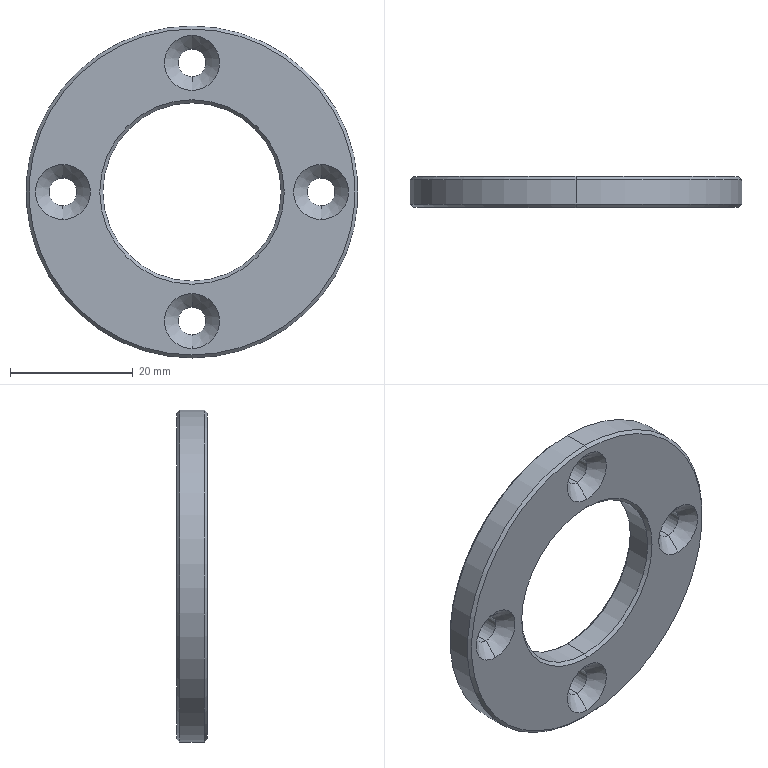Component | SolidWorks | ScrewRodBearingEndCap-1 | 1 solid | 30 faces | box 54 x 5 x 54 mm | volume 7578 mm3 | cone 16 | cylinder 12 | plane 2 | commonest cylinder face diameters 4.5 x8 29 x2 54 x2
build123d program:
from build123d import *

# Parameters (mm, degrees)
SKETCH1_R           = 27
SKETCH1_R_2         = 14.5
BOSS_EXTRUDE1_DEPTH = 5
CHAMFER1_SIZE       = 0.5
CIRPATTERN1_COUNT   = 4


with BuildPart() as part:
    # Sketch1 → Boss-Extrude1 (new body)
    with BuildSketch(Plane(origin=(0, 0, 0), x_dir=(1, 0, 0), z_dir=(0, 1, 0))):
        with Locations(Location((0, 0, 0), (0, 0, 270))):
            Circle(SKETCH1_R)
        with Locations(Location((0, 0, 0), (0, 0, 270))):
            Circle(SKETCH1_R_2, mode=Mode.SUBTRACT)
    extrude(amount=BOSS_EXTRUDE1_DEPTH)

    # Chamfer1
    chamfer1_edges = [part.edges().sort_by_distance(p)[0] for p in [
        (0, 0, -27),
        (0, 5, -27),
        (0, 0, -14.5),
        (0, 5, -14.5),
    ]]
    chamfer(chamfer1_edges, length=CHAMFER1_SIZE)

    # Sketch4 → M4 Hexagon Socket Countersunk Head Screw (revolve, cut)
    with BuildSketch(Plane(origin=(0, 0, 21), x_dir=(0, 0, -1), z_dir=(1, 0, 0))):
        Polygon((0, 0), (0, 16.352), (2.25, 15), (2.25, 2.23), (4.48, 0), align=None)
    m4_hexagon_socket_countersunk_head_screw = revolve(axis=Axis((0, -6.35, 21), (0, 1, 0)), mode=Mode.SUBTRACT)

    # CirPattern1: M4 Hexagon Socket Countersunk Head Screw ×4 about axis
    cirpattern1_axis = Axis((0, 0, 0), (0, 1, 0))
    for i in range(1, CIRPATTERN1_COUNT):
        add(m4_hexagon_socket_countersunk_head_screw.rotate(cirpattern1_axis, i * 360 / CIRPATTERN1_COUNT), mode=Mode.SUBTRACT)


solid = part.part

# Placed as in the assembly
solid = solid.moved(Location((-29.507, 212.589, 458), (0, 0, 0)))
STEP:
#1=COLOUR_RGB('',0.7922,0.8196,0.9333);
#2=FILL_AREA_STYLE_COLOUR('',#1);
#3=FILL_AREA_STYLE('',(#2));
#4=SURFACE_STYLE_FILL_AREA(#3);
#5=SURFACE_SIDE_STYLE('',(#4));
#6=SURFACE_STYLE_USAGE(.BOTH.,#5);
#7=PRESENTATION_STYLE_ASSIGNMENT((#6));
#8=CARTESIAN_POINT('',(-0.3349,8.457,18.12));
#9=VERTEX_POINT('',#8);
#10=CARTESIAN_POINT('',(-0.3349,8.457,17.943));
#11=VERTEX_POINT('',#10);
#12=CARTESIAN_POINT('',(-0.3349,8.457,18.031));
#13=DIRECTION('',(0.,-1.,0.));
#14=DIRECTION('',(0.,0.,-1.));
#15=AXIS2_PLACEMENT_3D('',#12,#13,#14);
#16=CIRCLE('',#15,0.08858);
#17=EDGE_CURVE('',#9,#11,#16,.T.);
#18=ORIENTED_EDGE('',*,*,#17,.F.);
#19=CARTESIAN_POINT('',(-0.3349,8.37,18.208));
#20=VERTEX_POINT('',#19);
#21=CARTESIAN_POINT('',(-0.3349,8.37,18.208));
#22=DIRECTION('',(0.,-0.7071,0.7071));
#23=VECTOR('',#22,39.37);
#24=LINE('',#21,#23);
#25=EDGE_CURVE('',#9,#20,#24,.T.);
#26=ORIENTED_EDGE('',*,*,#25,.T.);
#27=CARTESIAN_POINT('',(-0.3349,8.37,17.855));
#28=VERTEX_POINT('',#27);
#29=CARTESIAN_POINT('',(-0.3349,8.37,18.031));
#30=DIRECTION('',(0.,-1.,0.));
#31=DIRECTION('',(0.,0.,-1.));
#32=AXIS2_PLACEMENT_3D('',#29,#30,#31);
#33=CIRCLE('',#32,0.1764);
#34=EDGE_CURVE('',#20,#28,#33,.T.);
#35=ORIENTED_EDGE('',*,*,#34,.T.);
#36=CARTESIAN_POINT('',(-0.3349,8.37,17.855));
#37=DIRECTION('',(0.,-0.7071,-0.7071));
#38=VECTOR('',#37,39.37);
#39=LINE('',#36,#38);
#40=EDGE_CURVE('',#11,#28,#39,.T.);
#41=ORIENTED_EDGE('',*,*,#40,.F.);
#42=EDGE_LOOP('',(#18,#26,#35,#41));
#43=FACE_OUTER_BOUND('',#42,.T.);
#44=CARTESIAN_POINT('',(-0.3349,8.37,18.031));
#45=DIRECTION('',(0.,-1.,0.));
#46=DIRECTION('',(0.,0.,-1.));
#47=AXIS2_PLACEMENT_3D('',#44,#45,#46);
#48=CONICAL_SURFACE('',#47,0.1764,0.7854);
#49=ADVANCED_FACE('',(#43),#48,.F.);
#50=CARTESIAN_POINT('',(-0.3349,8.566,17.943));
#51=VERTEX_POINT('',#50);
#52=CARTESIAN_POINT('',(-0.3349,8.566,18.12));
#53=VERTEX_POINT('',#52);
#54=CARTESIAN_POINT('',(-0.3349,8.566,18.031));
#55=DIRECTION('',(0.,1.,0.));
#56=DIRECTION('',(0.,0.,1.));
#57=AXIS2_PLACEMENT_3D('',#54,#55,#56);
#58=CIRCLE('',#57,0.08858);
#59=EDGE_CURVE('',#51,#53,#58,.T.);
#60=ORIENTED_EDGE('',*,*,#59,.T.);
#61=CARTESIAN_POINT('',(-0.3349,8.37,18.12));
#62=DIRECTION('',(0.,-1.,0.));
#63=VECTOR('',#62,39.37);
#64=LINE('',#61,#63);
#65=EDGE_CURVE('',#53,#9,#64,.T.);
#66=ORIENTED_EDGE('',*,*,#65,.T.);
#67=ORIENTED_EDGE('',*,*,#17,.T.);
#68=CARTESIAN_POINT('',(-0.3349,8.37,17.943));
#69=DIRECTION('',(0.,-1.,0.));
#70=VECTOR('',#69,39.37);
#71=LINE('',#68,#70);
#72=EDGE_CURVE('',#51,#11,#71,.T.);
#73=ORIENTED_EDGE('',*,*,#72,.F.);
#74=EDGE_LOOP('',(#60,#66,#67,#73));
#75=FACE_OUTER_BOUND('',#74,.T.);
#76=CARTESIAN_POINT('',(-0.3349,8.37,18.031));
#77=DIRECTION('',(0.,-1.,0.));
#78=DIRECTION('',(0.,0.,-1.));
#79=AXIS2_PLACEMENT_3D('',#76,#77,#78);
#80=CYLINDRICAL_SURFACE('',#79,0.08858);
#81=ADVANCED_FACE('',(#75),#80,.F.);
#82=CARTESIAN_POINT('',(-1.162,8.457,17.293));
#83=VERTEX_POINT('',#82);
#84=CARTESIAN_POINT('',(-1.162,8.457,17.116));
#85=VERTEX_POINT('',#84);
#86=CARTESIAN_POINT('',(-1.162,8.457,17.205));
#87=DIRECTION('',(0.,-1.,0.));
#88=DIRECTION('',(0.,0.,-1.));
#89=AXIS2_PLACEMENT_3D('',#86,#87,#88);
#90=CIRCLE('',#89,0.08858);
#91=EDGE_CURVE('',#83,#85,#90,.T.);
#92=ORIENTED_EDGE('',*,*,#91,.F.);
#93=CARTESIAN_POINT('',(-1.162,8.37,17.381));
#94=VERTEX_POINT('',#93);
#95=CARTESIAN_POINT('',(-1.162,8.37,17.381));
#96=DIRECTION('',(0.,-0.7071,0.7071));
#97=VECTOR('',#96,39.37);
#98=LINE('',#95,#97);
#99=EDGE_CURVE('',#83,#94,#98,.T.);
#100=ORIENTED_EDGE('',*,*,#99,.T.);
#101=CARTESIAN_POINT('',(-1.162,8.37,17.028));
#102=VERTEX_POINT('',#101);
#103=CARTESIAN_POINT('',(-1.162,8.37,17.205));
#104=DIRECTION('',(0.,-1.,0.));
#105=DIRECTION('',(0.,0.,-1.));
#106=AXIS2_PLACEMENT_3D('',#103,#104,#105);
#107=CIRCLE('',#106,0.1764);
#108=EDGE_CURVE('',#94,#102,#107,.T.);
#109=ORIENTED_EDGE('',*,*,#108,.T.);
#110=CARTESIAN_POINT('',(-1.162,8.37,17.028));
#111=DIRECTION('',(0.,-0.7071,-0.7071));
#112=VECTOR('',#111,39.37);
#113=LINE('',#110,#112);
#114=EDGE_CURVE('',#85,#102,#113,.T.);
#115=ORIENTED_EDGE('',*,*,#114,.F.);
#116=EDGE_LOOP('',(#92,#100,#109,#115));
#117=FACE_OUTER_BOUND('',#116,.T.);
#118=CARTESIAN_POINT('',(-1.162,8.37,17.205));
#119=DIRECTION('',(0.,-1.,0.));
#120=DIRECTION('',(0.,0.,-1.));
#121=AXIS2_PLACEMENT_3D('',#118,#119,#120);
#122=CONICAL_SURFACE('',#121,0.1764,0.7854);
#123=ADVANCED_FACE('',(#117),#122,.F.);
#124=CARTESIAN_POINT('',(-1.162,8.566,17.116));
#125=VERTEX_POINT('',#124);
#126=CARTESIAN_POINT('',(-1.162,8.566,17.293));
#127=VERTEX_POINT('',#126);
#128=CARTESIAN_POINT('',(-1.162,8.566,17.205));
#129=DIRECTION('',(0.,1.,0.));
#130=DIRECTION('',(0.,0.,1.));
#131=AXIS2_PLACEMENT_3D('',#128,#129,#130);
#132=CIRCLE('',#131,0.08858);
#133=EDGE_CURVE('',#125,#127,#132,.T.);
#134=ORIENTED_EDGE('',*,*,#133,.T.);
#135=CARTESIAN_POINT('',(-1.162,8.37,17.293));
#136=DIRECTION('',(0.,-1.,0.));
#137=VECTOR('',#136,39.37);
#138=LINE('',#135,#137);
#139=EDGE_CURVE('',#127,#83,#138,.T.);
#140=ORIENTED_EDGE('',*,*,#139,.T.);
#141=ORIENTED_EDGE('',*,*,#91,.T.);
#142=CARTESIAN_POINT('',(-1.162,8.37,17.116));
#143=DIRECTION('',(0.,-1.,0.));
#144=VECTOR('',#143,39.37);
#145=LINE('',#142,#144);
#146=EDGE_CURVE('',#125,#85,#145,.T.);
#147=ORIENTED_EDGE('',*,*,#146,.F.);
#148=EDGE_LOOP('',(#134,#140,#141,#147));
#149=FACE_OUTER_BOUND('',#148,.T.);
#150=CARTESIAN_POINT('',(-1.162,8.37,17.205));
#151=DIRECTION('',(0.,-1.,0.));
#152=DIRECTION('',(0.,0.,-1.));
#153=AXIS2_PLACEMENT_3D('',#150,#151,#152);
#154=CYLINDRICAL_SURFACE('',#153,0.08858);
#155=ADVANCED_FACE('',(#149),#154,.F.);
#156=CARTESIAN_POINT('',(-1.988,8.457,18.12));
#157=VERTEX_POINT('',#156);
#158=CARTESIAN_POINT('',(-1.988,8.457,17.943));
#159=VERTEX_POINT('',#158);
#160=CARTESIAN_POINT('',(-1.988,8.457,18.031));
#161=DIRECTION('',(0.,-1.,0.));
#162=DIRECTION('',(0.,0.,-1.));
#163=AXIS2_PLACEMENT_3D('',#160,#161,#162);
#164=CIRCLE('',#163,0.08858);
#165=EDGE_CURVE('',#157,#159,#164,.T.);
#166=ORIENTED_EDGE('',*,*,#165,.F.);
#167=CARTESIAN_POINT('',(-1.988,8.37,18.208));
#168=VERTEX_POINT('',#167);
#169=CARTESIAN_POINT('',(-1.988,8.37,18.208));
#170=DIRECTION('',(0.,-0.7071,0.7071));
#171=VECTOR('',#170,39.37);
#172=LINE('',#169,#171);
#173=EDGE_CURVE('',#157,#168,#172,.T.);
#174=ORIENTED_EDGE('',*,*,#173,.T.);
#175=CARTESIAN_POINT('',(-1.988,8.37,17.855));
#176=VERTEX_POINT('',#175);
#177=CARTESIAN_POINT('',(-1.988,8.37,18.031));
#178=DIRECTION('',(0.,-1.,0.));
#179=DIRECTION('',(0.,0.,-1.));
#180=AXIS2_PLACEMENT_3D('',#177,#178,#179);
#181=CIRCLE('',#180,0.1764);
#182=EDGE_CURVE('',#168,#176,#181,.T.);
#183=ORIENTED_EDGE('',*,*,#182,.T.);
#184=CARTESIAN_POINT('',(-1.988,8.37,17.855));
#185=DIRECTION('',(0.,-0.7071,-0.7071));
#186=VECTOR('',#185,39.37);
#187=LINE('',#184,#186);
#188=EDGE_CURVE('',#159,#176,#187,.T.);
#189=ORIENTED_EDGE('',*,*,#188,.F.);
#190=EDGE_LOOP('',(#166,#174,#183,#189));
#191=FACE_OUTER_BOUND('',#190,.T.);
#192=CARTESIAN_POINT('',(-1.988,8.37,18.031));
#193=DIRECTION('',(0.,-1.,0.));
#194=DIRECTION('',(0.,0.,-1.));
#195=AXIS2_PLACEMENT_3D('',#192,#193,#194);
#196=CONICAL_SURFACE('',#195,0.1764,0.7854);
#197=ADVANCED_FACE('',(#191),#196,.F.);
#198=CARTESIAN_POINT('',(-1.988,8.566,17.943));
#199=VERTEX_POINT('',#198);
#200=CARTESIAN_POINT('',(-1.988,8.566,18.12));
#201=VERTEX_POINT('',#200);
#202=CARTESIAN_POINT('',(-1.988,8.566,18.031));
#203=DIRECTION('',(0.,1.,0.));
#204=DIRECTION('',(0.,0.,1.));
#205=AXIS2_PLACEMENT_3D('',#202,#203,#204);
#206=CIRCLE('',#205,0.08858);
#207=EDGE_CURVE('',#199,#201,#206,.T.);
#208=ORIENTED_EDGE('',*,*,#207,.T.);
#209=CARTESIAN_POINT('',(-1.988,8.37,18.12));
#210=DIRECTION('',(0.,-1.,0.));
#211=VECTOR('',#210,39.37);
#212=LINE('',#209,#211);
#213=EDGE_CURVE('',#201,#157,#212,.T.);
#214=ORIENTED_EDGE('',*,*,#213,.T.);
#215=ORIENTED_EDGE('',*,*,#165,.T.);
#216=CARTESIAN_POINT('',(-1.988,8.37,17.943));
#217=DIRECTION('',(0.,-1.,0.));
#218=VECTOR('',#217,39.37);
#219=LINE('',#216,#218);
#220=EDGE_CURVE('',#199,#159,#219,.T.);
#221=ORIENTED_EDGE('',*,*,#220,.F.);
#222=EDGE_LOOP('',(#208,#214,#215,#221));
#223=FACE_OUTER_BOUND('',#222,.T.);
#224=CARTESIAN_POINT('',(-1.988,8.37,18.031));
#225=DIRECTION('',(0.,-1.,0.));
#226=DIRECTION('',(0.,0.,-1.));
#227=AXIS2_PLACEMENT_3D('',#224,#225,#226);
#228=CYLINDRICAL_SURFACE('',#227,0.08858);
#229=ADVANCED_FACE('',(#223),#228,.F.);
#230=CARTESIAN_POINT('',(-1.162,8.457,18.947));
#231=VERTEX_POINT('',#230);
#232=CARTESIAN_POINT('',(-1.162,8.457,18.77));
#233=VERTEX_POINT('',#232);
#234=CARTESIAN_POINT('',(-1.162,8.457,18.858));
#235=DIRECTION('',(0.,-1.,0.));
#236=DIRECTION('',(0.,0.,-1.));
#237=AXIS2_PLACEMENT_3D('',#234,#235,#236);
#238=CIRCLE('',#237,0.08858);
#239=EDGE_CURVE('',#231,#233,#238,.T.);
#240=ORIENTED_EDGE('',*,*,#239,.F.);
#241=CARTESIAN_POINT('',(-1.162,8.37,19.035));
#242=VERTEX_POINT('',#241);
#243=CARTESIAN_POINT('',(-1.162,8.37,19.035));
#244=DIRECTION('',(0.,-0.7071,0.7071));
#245=VECTOR('',#244,39.37);
#246=LINE('',#243,#245);
#247=EDGE_CURVE('',#231,#242,#246,.T.);
#248=ORIENTED_EDGE('',*,*,#247,.T.);
#249=CARTESIAN_POINT('',(-1.162,8.37,18.682));
#250=VERTEX_POINT('',#249);
#251=CARTESIAN_POINT('',(-1.162,8.37,18.858));
#252=DIRECTION('',(0.,-1.,0.));
#253=DIRECTION('',(0.,0.,-1.));
#254=AXIS2_PLACEMENT_3D('',#251,#252,#253);
#255=CIRCLE('',#254,0.1764);
#256=EDGE_CURVE('',#242,#250,#255,.T.);
#257=ORIENTED_EDGE('',*,*,#256,.T.);
#258=CARTESIAN_POINT('',(-1.162,8.37,18.682));
#259=DIRECTION('',(0.,-0.7071,-0.7071));
#260=VECTOR('',#259,39.37);
#261=LINE('',#258,#260);
#262=EDGE_CURVE('',#233,#250,#261,.T.);
#263=ORIENTED_EDGE('',*,*,#262,.F.);
#264=EDGE_LOOP('',(#240,#248,#257,#263));
#265=FACE_OUTER_BOUND('',#264,.T.);
#266=CARTESIAN_POINT('',(-1.162,8.37,18.858));
#267=DIRECTION('',(0.,-1.,0.));
#268=DIRECTION('',(0.,0.,-1.));
#269=AXIS2_PLACEMENT_3D('',#266,#267,#268);
#270=CONICAL_SURFACE('',#269,0.1764,0.7854);
#271=ADVANCED_FACE('',(#265),#270,.F.);
#272=CARTESIAN_POINT('',(-1.162,8.566,18.77));
#273=VERTEX_POINT('',#272);
#274=CARTESIAN_POINT('',(-1.162,8.566,18.947));
#275=VERTEX_POINT('',#274);
#276=CARTESIAN_POINT('',(-1.162,8.566,18.858));
#277=DIRECTION('',(0.,1.,0.));
#278=DIRECTION('',(0.,0.,1.));
#279=AXIS2_PLACEMENT_3D('',#276,#277,#278);
#280=CIRCLE('',#279,0.08858);
#281=EDGE_CURVE('',#273,#275,#280,.T.);
#282=ORIENTED_EDGE('',*,*,#281,.T.);
#283=CARTESIAN_POINT('',(-1.162,8.37,18.947));
#284=DIRECTION('',(0.,-1.,0.));
#285=VECTOR('',#284,39.37);
#286=LINE('',#283,#285);
#287=EDGE_CURVE('',#275,#231,#286,.T.);
#288=ORIENTED_EDGE('',*,*,#287,.T.);
#289=ORIENTED_EDGE('',*,*,#239,.T.);
#290=CARTESIAN_POINT('',(-1.162,8.37,18.77));
#291=DIRECTION('',(0.,-1.,0.));
#292=VECTOR('',#291,39.37);
#293=LINE('',#290,#292);
#294=EDGE_CURVE('',#273,#233,#293,.T.);
#295=ORIENTED_EDGE('',*,*,#294,.F.);
#296=EDGE_LOOP('',(#282,#288,#289,#295));
#297=FACE_OUTER_BOUND('',#296,.T.);
#298=CARTESIAN_POINT('',(-1.162,8.37,18.858));
#299=DIRECTION('',(0.,-1.,0.));
#300=DIRECTION('',(0.,0.,-1.));
#301=AXIS2_PLACEMENT_3D('',#298,#299,#300);
#302=CYLINDRICAL_SURFACE('',#301,0.08858);
#303=ADVANCED_FACE('',(#297),#302,.F.);
#304=CARTESIAN_POINT('',(-1.162,8.547,17.461));
#305=VERTEX_POINT('',#304);
#306=CARTESIAN_POINT('',(-1.162,8.547,18.602));
#307=VERTEX_POINT('',#306);
#308=CARTESIAN_POINT('',(-1.162,8.547,18.031));
#309=DIRECTION('',(0.,1.,0.));
#310=DIRECTION('',(0.,0.,1.));
#311=AXIS2_PLACEMENT_3D('',#308,#309,#310);
#312=CIRCLE('',#311,0.5709);
#313=EDGE_CURVE('',#305,#307,#312,.T.);
#314=ORIENTED_EDGE('',*,*,#313,.F.);
#315=CARTESIAN_POINT('',(-1.162,8.566,17.441));
#316=VERTEX_POINT('',#315);
#317=CARTESIAN_POINT('',(-1.162,8.547,17.461));
#318=DIRECTION('',(0.,0.7071,-0.7071));
#319=VECTOR('',#318,39.37);
#320=LINE('',#317,#319);
#321=EDGE_CURVE('',#305,#316,#320,.T.);
#322=ORIENTED_EDGE('',*,*,#321,.T.);
#323=CARTESIAN_POINT('',(-1.162,8.566,18.622));
#324=VERTEX_POINT('',#323);
#325=CARTESIAN_POINT('',(-1.162,8.566,18.031));
#326=DIRECTION('',(0.,-1.,0.));
#327=DIRECTION('',(0.,0.,1.));
#328=AXIS2_PLACEMENT_3D('',#325,#326,#327);
#329=CIRCLE('',#328,0.5906);
#330=EDGE_CURVE('',#324,#316,#329,.T.);
#331=ORIENTED_EDGE('',*,*,#330,.F.);
#332=CARTESIAN_POINT('',(-1.162,8.547,18.602));
#333=DIRECTION('',(0.,0.7071,0.7071));
#334=VECTOR('',#333,39.37);
#335=LINE('',#332,#334);
#336=EDGE_CURVE('',#307,#324,#335,.T.);
#337=ORIENTED_EDGE('',*,*,#336,.F.);
#338=EDGE_LOOP('',(#314,#322,#331,#337));
#339=FACE_OUTER_BOUND('',#338,.T.);
#340=CARTESIAN_POINT('',(-1.162,8.547,18.031));
#341=DIRECTION('',(0.,1.,0.));
#342=DIRECTION('',(0.,0.,1.));
#343=AXIS2_PLACEMENT_3D('',#340,#341,#342);
#344=CONICAL_SURFACE('',#343,0.5709,0.7854);
#345=ADVANCED_FACE('',(#339),#344,.F.);
#346=CARTESIAN_POINT('',(-1.162,8.566,19.075));
#347=VERTEX_POINT('',#346);
#348=CARTESIAN_POINT('',(-1.162,8.566,16.988));
#349=VERTEX_POINT('',#348);
#350=CARTESIAN_POINT('',(-1.162,8.566,18.031));
#351=DIRECTION('',(0.,1.,0.));
#352=DIRECTION('',(0.,0.,1.));
#353=AXIS2_PLACEMENT_3D('',#350,#351,#352);
#354=CIRCLE('',#353,1.043);
#355=EDGE_CURVE('',#347,#349,#354,.T.);
#356=ORIENTED_EDGE('',*,*,#355,.F.);
#357=CARTESIAN_POINT('',(-1.162,8.547,19.094));
#358=VERTEX_POINT('',#357);
#359=CARTESIAN_POINT('',(-1.162,8.566,19.075));
#360=DIRECTION('',(0.,-0.7071,0.7071));
#361=VECTOR('',#360,39.37);
#362=LINE('',#359,#361);
#363=EDGE_CURVE('',#347,#358,#362,.T.);
#364=ORIENTED_EDGE('',*,*,#363,.T.);
#365=CARTESIAN_POINT('',(-1.162,8.547,16.969));
#366=VERTEX_POINT('',#365);
#367=CARTESIAN_POINT('',(-1.162,8.547,18.031));
#368=DIRECTION('',(0.,-1.,0.));
#369=DIRECTION('',(0.,0.,1.));
#370=AXIS2_PLACEMENT_3D('',#367,#368,#369);
#371=CIRCLE('',#370,1.063);
#372=EDGE_CURVE('',#366,#358,#371,.T.);
#373=ORIENTED_EDGE('',*,*,#372,.F.);
#374=CARTESIAN_POINT('',(-1.162,8.566,16.988));
#375=DIRECTION('',(0.,-0.7071,-0.7071));
#376=VECTOR('',#375,39.37);
#377=LINE('',#374,#376);
#378=EDGE_CURVE('',#349,#366,#377,.T.);
#379=ORIENTED_EDGE('',*,*,#378,.F.);
#380=EDGE_LOOP('',(#356,#364,#373,#379));
#381=FACE_OUTER_BOUND('',#380,.T.);
#382=CARTESIAN_POINT('',(-1.162,8.566,18.031));
#383=DIRECTION('',(0.,-1.,0.));
#384=DIRECTION('',(0.,0.,-1.));
#385=AXIS2_PLACEMENT_3D('',#382,#383,#384);
#386=CONICAL_SURFACE('',#385,1.043,0.7854);
#387=ADVANCED_FACE('',(#381),#386,.T.);
#388=CARTESIAN_POINT('',(-1.162,8.37,16.988));
#389=VERTEX_POINT('',#388);
#390=CARTESIAN_POINT('',(-1.162,8.37,19.075));
#391=VERTEX_POINT('',#390);
#392=CARTESIAN_POINT('',(-1.162,8.37,18.031));
#393=DIRECTION('',(0.,-1.,0.));
#394=DIRECTION('',(0.,0.,1.));
#395=AXIS2_PLACEMENT_3D('',#392,#393,#394);
#396=CIRCLE('',#395,1.043);
#397=EDGE_CURVE('',#389,#391,#396,.T.);
#398=ORIENTED_EDGE('',*,*,#397,.F.);
#399=CARTESIAN_POINT('',(-1.162,8.389,16.969));
#400=VERTEX_POINT('',#399);
#401=CARTESIAN_POINT('',(-1.162,8.389,16.969));
#402=DIRECTION('',(0.,0.7071,-0.7071));
#403=VECTOR('',#402,39.37);
#404=LINE('',#401,#403);
#405=EDGE_CURVE('',#389,#400,#404,.T.);
#406=ORIENTED_EDGE('',*,*,#405,.T.);
#407=CARTESIAN_POINT('',(-1.162,8.389,19.094));
#408=VERTEX_POINT('',#407);
#409=CARTESIAN_POINT('',(-1.162,8.389,18.031));
#410=DIRECTION('',(0.,1.,0.));
#411=DIRECTION('',(0.,0.,1.));
#412=AXIS2_PLACEMENT_3D('',#409,#410,#411);
#413=CIRCLE('',#412,1.063);
#414=EDGE_CURVE('',#408,#400,#413,.T.);
#415=ORIENTED_EDGE('',*,*,#414,.F.);
#416=CARTESIAN_POINT('',(-1.162,8.389,19.094));
#417=DIRECTION('',(0.,0.7071,0.7071));
#418=VECTOR('',#417,39.37);
#419=LINE('',#416,#418);
#420=EDGE_CURVE('',#391,#408,#419,.T.);
#421=ORIENTED_EDGE('',*,*,#420,.F.);
#422=EDGE_LOOP('',(#398,#406,#415,#421));
#423=FACE_OUTER_BOUND('',#422,.T.);
#424=CARTESIAN_POINT('',(-1.162,8.389,18.031));
#425=DIRECTION('',(0.,1.,0.));
#426=DIRECTION('',(0.,0.,1.));
#427=AXIS2_PLACEMENT_3D('',#424,#425,#426);
#428=CONICAL_SURFACE('',#427,1.063,0.7854);
#429=ADVANCED_FACE('',(#423),#428,.T.);
#430=CARTESIAN_POINT('',(-1.162,8.389,18.602));
#431=VERTEX_POINT('',#430);
#432=CARTESIAN_POINT('',(-1.162,8.389,17.461));
#433=VERTEX_POINT('',#432);
#434=CARTESIAN_POINT('',(-1.162,8.389,18.031));
#435=DIRECTION('',(0.,-1.,0.));
#436=DIRECTION('',(0.,0.,1.));
#437=AXIS2_PLACEMENT_3D('',#434,#435,#436);
#438=CIRCLE('',#437,0.5709);
#439=EDGE_CURVE('',#431,#433,#438,.T.);
#440=ORIENTED_EDGE('',*,*,#439,.F.);
#441=CARTESIAN_POINT('',(-1.162,8.37,18.622));
#442=VERTEX_POINT('',#441);
#443=CARTESIAN_POINT('',(-1.162,8.37,18.622));
#444=DIRECTION('',(0.,-0.7071,0.7071));
#445=VECTOR('',#444,39.37);
#446=LINE('',#443,#445);
#447=EDGE_CURVE('',#431,#442,#446,.T.);
#448=ORIENTED_EDGE('',*,*,#447,.T.);
#449=CARTESIAN_POINT('',(-1.162,8.37,17.441));
#450=VERTEX_POINT('',#449);
#451=CARTESIAN_POINT('',(-1.162,8.37,18.031));
#452=DIRECTION('',(0.,1.,0.));
#453=DIRECTION('',(0.,0.,1.));
#454=AXIS2_PLACEMENT_3D('',#451,#452,#453);
#455=CIRCLE('',#454,0.5906);
#456=EDGE_CURVE('',#450,#442,#455,.T.);
#457=ORIENTED_EDGE('',*,*,#456,.F.);
#458=CARTESIAN_POINT('',(-1.162,8.37,17.441));
#459=DIRECTION('',(0.,-0.7071,-0.7071));
#460=VECTOR('',#459,39.37);
#461=LINE('',#458,#460);
#462=EDGE_CURVE('',#433,#450,#461,.T.);
#463=ORIENTED_EDGE('',*,*,#462,.F.);
#464=EDGE_LOOP('',(#440,#448,#457,#463));
#465=FACE_OUTER_BOUND('',#464,.T.);
#466=CARTESIAN_POINT('',(-1.162,8.37,18.031));
#467=DIRECTION('',(0.,-1.,0.));
#468=DIRECTION('',(0.,0.,-1.));
#469=AXIS2_PLACEMENT_3D('',#466,#467,#468);
#470=CONICAL_SURFACE('',#469,0.5906,0.7854);
#471=ADVANCED_FACE('',(#465),#470,.F.);
#472=ORIENTED_EDGE('',*,*,#313,.T.);
#473=CARTESIAN_POINT('',(-1.162,8.566,18.602));
#474=DIRECTION('',(0.,-1.,0.));
#475=VECTOR('',#474,39.37);
#476=LINE('',#473,#475);
#477=EDGE_CURVE('',#307,#431,#476,.T.);
#478=ORIENTED_EDGE('',*,*,#477,.T.);
#479=ORIENTED_EDGE('',*,*,#439,.T.);
#480=CARTESIAN_POINT('',(-1.162,8.566,17.461));
#481=DIRECTION('',(0.,-1.,0.));
#482=VECTOR('',#481,39.37);
#483=LINE('',#480,#482);
#484=EDGE_CURVE('',#305,#433,#483,.T.);
#485=ORIENTED_EDGE('',*,*,#484,.F.);
#486=EDGE_LOOP('',(#472,#478,#479,#485));
#487=FACE_OUTER_BOUND('',#486,.T.);
#488=CARTESIAN_POINT('',(-1.162,8.566,18.031));
#489=DIRECTION('',(0.,-1.,0.));
#490=DIRECTION('',(0.,0.,-1.));
#491=AXIS2_PLACEMENT_3D('',#488,#489,#490);
#492=CYLINDRICAL_SURFACE('',#491,0.5709);
#493=ADVANCED_FACE('',(#487),#492,.F.);
#494=ORIENTED_EDGE('',*,*,#372,.T.);
#495=CARTESIAN_POINT('',(-1.162,8.566,19.094));
#496=DIRECTION('',(0.,-1.,0.));
#497=VECTOR('',#496,39.37);
#498=LINE('',#495,#497);
#499=EDGE_CURVE('',#358,#408,#498,.T.);
#500=ORIENTED_EDGE('',*,*,#499,.T.);
#501=ORIENTED_EDGE('',*,*,#414,.T.);
#502=CARTESIAN_POINT('',(-1.162,8.566,16.969));
#503=DIRECTION('',(0.,-1.,0.));
#504=VECTOR('',#503,39.37);
#505=LINE('',#502,#504);
#506=EDGE_CURVE('',#366,#400,#505,.T.);
#507=ORIENTED_EDGE('',*,*,#506,.F.);
#508=EDGE_LOOP('',(#494,#500,#501,#507));
#509=FACE_OUTER_BOUND('',#508,.T.);
#510=CARTESIAN_POINT('',(-1.162,8.566,18.031));
#511=DIRECTION('',(0.,-1.,0.));
#512=DIRECTION('',(0.,0.,-1.));
#513=AXIS2_PLACEMENT_3D('',#510,#511,#512);
#514=CYLINDRICAL_SURFACE('',#513,1.063);
#515=ADVANCED_FACE('',(#509),#514,.T.);
#516=ORIENTED_EDGE('',*,*,#59,.F.);
#517=CARTESIAN_POINT('',(-0.3349,8.566,18.031));
#518=DIRECTION('',(0.,1.,0.));
#519=DIRECTION('',(0.,0.,1.));
#520=AXIS2_PLACEMENT_3D('',#517,#518,#519);
#521=CIRCLE('',#520,0.08858);
#522=EDGE_CURVE('',#53,#51,#521,.T.);
#523=ORIENTED_EDGE('',*,*,#522,.F.);
#524=EDGE_LOOP('',(#516,#523));
#525=FACE_BOUND('',#524,.T.);
#526=ORIENTED_EDGE('',*,*,#133,.F.);
#527=CARTESIAN_POINT('',(-1.162,8.566,17.205));
#528=DIRECTION('',(0.,1.,0.));
#529=DIRECTION('',(0.,0.,1.));
#530=AXIS2_PLACEMENT_3D('',#527,#528,#529);
#531=CIRCLE('',#530,0.08858);
#532=EDGE_CURVE('',#127,#125,#531,.T.);
#533=ORIENTED_EDGE('',*,*,#532,.F.);
#534=EDGE_LOOP('',(#526,#533));
#535=FACE_BOUND('',#534,.T.);
#536=ORIENTED_EDGE('',*,*,#207,.F.);
#537=CARTESIAN_POINT('',(-1.988,8.566,18.031));
#538=DIRECTION('',(0.,1.,0.));
#539=DIRECTION('',(0.,0.,1.));
#540=AXIS2_PLACEMENT_3D('',#537,#538,#539);
#541=CIRCLE('',#540,0.08858);
#542=EDGE_CURVE('',#201,#199,#541,.T.);
#543=ORIENTED_EDGE('',*,*,#542,.F.);
#544=EDGE_LOOP('',(#536,#543));
#545=FACE_BOUND('',#544,.T.);
#546=ORIENTED_EDGE('',*,*,#281,.F.);
#547=CARTESIAN_POINT('',(-1.162,8.566,18.858));
#548=DIRECTION('',(0.,1.,0.));
#549=DIRECTION('',(0.,0.,1.));
#550=AXIS2_PLACEMENT_3D('',#547,#548,#549);
#551=CIRCLE('',#550,0.08858);
#552=EDGE_CURVE('',#275,#273,#551,.T.);
#553=ORIENTED_EDGE('',*,*,#552,.F.);
#554=EDGE_LOOP('',(#546,#553));
#555=FACE_BOUND('',#554,.T.);
#556=CARTESIAN_POINT('',(-1.162,8.566,18.031));
#557=DIRECTION('',(0.,1.,0.));
#558=DIRECTION('',(0.,0.,1.));
#559=AXIS2_PLACEMENT_3D('',#556,#557,#558);
#560=CIRCLE('',#559,1.043);
#561=EDGE_CURVE('',#349,#347,#560,.T.);
#562=ORIENTED_EDGE('',*,*,#561,.T.);
#563=ORIENTED_EDGE('',*,*,#355,.T.);
#564=EDGE_LOOP('',(#562,#563));
#565=FACE_OUTER_BOUND('',#564,.T.);
#566=ORIENTED_EDGE('',*,*,#330,.T.);
#567=CARTESIAN_POINT('',(-1.162,8.566,18.031));
#568=DIRECTION('',(0.,-1.,0.));
#569=DIRECTION('',(0.,0.,1.));
#570=AXIS2_PLACEMENT_3D('',#567,#568,#569);
#571=CIRCLE('',#570,0.5906);
#572=EDGE_CURVE('',#316,#324,#571,.T.);
#573=ORIENTED_EDGE('',*,*,#572,.T.);
#574=EDGE_LOOP('',(#566,#573));
#575=FACE_BOUND('',#574,.T.);
#576=CARTESIAN_POINT('',(-1.162,8.566,18.031));
#577=DIRECTION('',(0.,1.,0.));
#578=DIRECTION('',(0.,0.,1.));
#579=AXIS2_PLACEMENT_3D('',#576,#577,#578);
#580=PLANE('',#579);
#581=ADVANCED_FACE('',(#525,#535,#545,#555,#565,#575),#580,.T.);
#582=CARTESIAN_POINT('',(-0.3349,8.37,18.031));
#583=DIRECTION('',(0.,-1.,0.));
#584=DIRECTION('',(0.,0.,-1.));
#585=AXIS2_PLACEMENT_3D('',#582,#583,#584);
#586=CIRCLE('',#585,0.1764);
#587=EDGE_CURVE('',#28,#20,#586,.T.);
#588=ORIENTED_EDGE('',*,*,#587,.F.);
#589=ORIENTED_EDGE('',*,*,#34,.F.);
#590=EDGE_LOOP('',(#588,#589));
#591=FACE_BOUND('',#590,.T.);
#592=CARTESIAN_POINT('',(-1.162,8.37,17.205));
#593=DIRECTION('',(0.,-1.,0.));
#594=DIRECTION('',(0.,0.,-1.));
#595=AXIS2_PLACEMENT_3D('',#592,#593,#594);
#596=CIRCLE('',#595,0.1764);
#597=EDGE_CURVE('',#102,#94,#596,.T.);
#598=ORIENTED_EDGE('',*,*,#597,.F.);
#599=ORIENTED_EDGE('',*,*,#108,.F.);
#600=EDGE_LOOP('',(#598,#599));
#601=FACE_BOUND('',#600,.T.);
#602=CARTESIAN_POINT('',(-1.988,8.37,18.031));
#603=DIRECTION('',(0.,-1.,0.));
#604=DIRECTION('',(0.,0.,-1.));
#605=AXIS2_PLACEMENT_3D('',#602,#603,#604);
#606=CIRCLE('',#605,0.1764);
#607=EDGE_CURVE('',#176,#168,#606,.T.);
#608=ORIENTED_EDGE('',*,*,#607,.F.);
#609=ORIENTED_EDGE('',*,*,#182,.F.);
#610=EDGE_LOOP('',(#608,#609));
#611=FACE_BOUND('',#610,.T.);
#612=CARTESIAN_POINT('',(-1.162,8.37,18.858));
#613=DIRECTION('',(0.,-1.,0.));
#614=DIRECTION('',(0.,0.,-1.));
#615=AXIS2_PLACEMENT_3D('',#612,#613,#614);
#616=CIRCLE('',#615,0.1764);
#617=EDGE_CURVE('',#250,#242,#616,.T.);
#618=ORIENTED_EDGE('',*,*,#617,.F.);
#619=ORIENTED_EDGE('',*,*,#256,.F.);
#620=EDGE_LOOP('',(#618,#619));
#621=FACE_BOUND('',#620,.T.);
#622=ORIENTED_EDGE('',*,*,#456,.T.);
#623=CARTESIAN_POINT('',(-1.162,8.37,18.031));
#624=DIRECTION('',(0.,1.,0.));
#625=DIRECTION('',(0.,0.,1.));
#626=AXIS2_PLACEMENT_3D('',#623,#624,#625);
#627=CIRCLE('',#626,0.5906);
#628=EDGE_CURVE('',#442,#450,#627,.T.);
#629=ORIENTED_EDGE('',*,*,#628,.T.);
#630=EDGE_LOOP('',(#622,#629));
#631=FACE_BOUND('',#630,.T.);
#632=CARTESIAN_POINT('',(-1.162,8.37,18.031));
#633=DIRECTION('',(0.,-1.,0.));
#634=DIRECTION('',(0.,0.,1.));
#635=AXIS2_PLACEMENT_3D('',#632,#633,#634);
#636=CIRCLE('',#635,1.043);
#637=EDGE_CURVE('',#391,#389,#636,.T.);
#638=ORIENTED_EDGE('',*,*,#637,.T.);
#639=ORIENTED_EDGE('',*,*,#397,.T.);
#640=EDGE_LOOP('',(#638,#639));
#641=FACE_OUTER_BOUND('',#640,.T.);
#642=CARTESIAN_POINT('',(-1.162,8.37,18.031));
#643=DIRECTION('',(0.,1.,0.));
#644=DIRECTION('',(0.,0.,1.));
#645=AXIS2_PLACEMENT_3D('',#642,#643,#644);
#646=PLANE('',#645);
#647=ADVANCED_FACE('',(#591,#601,#611,#621,#631,#641),#646,.F.);
#648=ORIENTED_EDGE('',*,*,#499,.F.);
#649=CARTESIAN_POINT('',(-1.162,8.547,18.031));
#650=DIRECTION('',(0.,-1.,0.));
#651=DIRECTION('',(0.,0.,1.));
#652=AXIS2_PLACEMENT_3D('',#649,#650,#651);
#653=CIRCLE('',#652,1.063);
#654=EDGE_CURVE('',#358,#366,#653,.T.);
#655=ORIENTED_EDGE('',*,*,#654,.T.);
#656=ORIENTED_EDGE('',*,*,#506,.T.);
#657=CARTESIAN_POINT('',(-1.162,8.389,18.031));
#658=DIRECTION('',(0.,1.,0.));
#659=DIRECTION('',(0.,0.,1.));
#660=AXIS2_PLACEMENT_3D('',#657,#658,#659);
#661=CIRCLE('',#660,1.063);
#662=EDGE_CURVE('',#400,#408,#661,.T.);
#663=ORIENTED_EDGE('',*,*,#662,.T.);
#664=EDGE_LOOP('',(#648,#655,#656,#663));
#665=FACE_OUTER_BOUND('',#664,.T.);
#666=CARTESIAN_POINT('',(-1.162,8.566,18.031));
#667=DIRECTION('',(0.,-1.,0.));
#668=DIRECTION('',(0.,0.,-1.));
#669=AXIS2_PLACEMENT_3D('',#666,#667,#668);
#670=CYLINDRICAL_SURFACE('',#669,1.063);
#671=ADVANCED_FACE('',(#665),#670,.T.);
#672=ORIENTED_EDGE('',*,*,#477,.F.);
#673=CARTESIAN_POINT('',(-1.162,8.547,18.031));
#674=DIRECTION('',(0.,1.,0.));
#675=DIRECTION('',(0.,0.,1.));
#676=AXIS2_PLACEMENT_3D('',#673,#674,#675);
#677=CIRCLE('',#676,0.5709);
#678=EDGE_CURVE('',#307,#305,#677,.T.);
#679=ORIENTED_EDGE('',*,*,#678,.T.);
#680=ORIENTED_EDGE('',*,*,#484,.T.);
#681=CARTESIAN_POINT('',(-1.162,8.389,18.031));
#682=DIRECTION('',(0.,-1.,0.));
#683=DIRECTION('',(0.,0.,1.));
#684=AXIS2_PLACEMENT_3D('',#681,#682,#683);
#685=CIRCLE('',#684,0.5709);
#686=EDGE_CURVE('',#433,#431,#685,.T.);
#687=ORIENTED_EDGE('',*,*,#686,.T.);
#688=EDGE_LOOP('',(#672,#679,#680,#687));
#689=FACE_OUTER_BOUND('',#688,.T.);
#690=CARTESIAN_POINT('',(-1.162,8.566,18.031));
#691=DIRECTION('',(0.,-1.,0.));
#692=DIRECTION('',(0.,0.,-1.));
#693=AXIS2_PLACEMENT_3D('',#690,#691,#692);
#694=CYLINDRICAL_SURFACE('',#693,0.5709);
#695=ADVANCED_FACE('',(#689),#694,.F.);
#696=ORIENTED_EDGE('',*,*,#447,.F.);
#697=ORIENTED_EDGE('',*,*,#686,.F.);
#698=ORIENTED_EDGE('',*,*,#462,.T.);
#699=ORIENTED_EDGE('',*,*,#628,.F.);
#700=EDGE_LOOP('',(#696,#697,#698,#699));
#701=FACE_OUTER_BOUND('',#700,.T.);
#702=CARTESIAN_POINT('',(-1.162,8.37,18.031));
#703=DIRECTION('',(0.,-1.,0.));
#704=DIRECTION('',(0.,0.,-1.));
#705=AXIS2_PLACEMENT_3D('',#702,#703,#704);
#706=CONICAL_SURFACE('',#705,0.5906,0.7854);
#707=ADVANCED_FACE('',(#701),#706,.F.);
#708=ORIENTED_EDGE('',*,*,#405,.F.);
#709=ORIENTED_EDGE('',*,*,#637,.F.);
#710=ORIENTED_EDGE('',*,*,#420,.T.);
#711=ORIENTED_EDGE('',*,*,#662,.F.);
#712=EDGE_LOOP('',(#708,#709,#710,#711));
#713=FACE_OUTER_BOUND('',#712,.T.);
#714=CARTESIAN_POINT('',(-1.162,8.389,18.031));
#715=DIRECTION('',(0.,1.,0.));
#716=DIRECTION('',(0.,0.,1.));
#717=AXIS2_PLACEMENT_3D('',#714,#715,#716);
#718=CONICAL_SURFACE('',#717,1.063,0.7854);
#719=ADVANCED_FACE('',(#713),#718,.T.);
#720=ORIENTED_EDGE('',*,*,#363,.F.);
#721=ORIENTED_EDGE('',*,*,#561,.F.);
#722=ORIENTED_EDGE('',*,*,#378,.T.);
#723=ORIENTED_EDGE('',*,*,#654,.F.);
#724=EDGE_LOOP('',(#720,#721,#722,#723));
#725=FACE_OUTER_BOUND('',#724,.T.);
#726=CARTESIAN_POINT('',(-1.162,8.566,18.031));
#727=DIRECTION('',(0.,-1.,0.));
#728=DIRECTION('',(0.,0.,-1.));
#729=AXIS2_PLACEMENT_3D('',#726,#727,#728);
#730=CONICAL_SURFACE('',#729,1.043,0.7854);
#731=ADVANCED_FACE('',(#725),#730,.T.);
#732=ORIENTED_EDGE('',*,*,#321,.F.);
#733=ORIENTED_EDGE('',*,*,#678,.F.);
#734=ORIENTED_EDGE('',*,*,#336,.T.);
#735=ORIENTED_EDGE('',*,*,#572,.F.);
#736=EDGE_LOOP('',(#732,#733,#734,#735));
#737=FACE_OUTER_BOUND('',#736,.T.);
#738=CARTESIAN_POINT('',(-1.162,8.547,18.031));
#739=DIRECTION('',(0.,1.,0.));
#740=DIRECTION('',(0.,0.,1.));
#741=AXIS2_PLACEMENT_3D('',#738,#739,#740);
#742=CONICAL_SURFACE('',#741,0.5709,0.7854);
#743=ADVANCED_FACE('',(#737),#742,.F.);
#744=ORIENTED_EDGE('',*,*,#287,.F.);
#745=ORIENTED_EDGE('',*,*,#552,.T.);
#746=ORIENTED_EDGE('',*,*,#294,.T.);
#747=CARTESIAN_POINT('',(-1.162,8.457,18.858));
#748=DIRECTION('',(0.,-1.,0.));
#749=DIRECTION('',(0.,0.,-1.));
#750=AXIS2_PLACEMENT_3D('',#747,#748,#749);
#751=CIRCLE('',#750,0.08858);
#752=EDGE_CURVE('',#233,#231,#751,.T.);
#753=ORIENTED_EDGE('',*,*,#752,.T.);
#754=EDGE_LOOP('',(#744,#745,#746,#753));
#755=FACE_OUTER_BOUND('',#754,.T.);
#756=CARTESIAN_POINT('',(-1.162,8.37,18.858));
#757=DIRECTION('',(0.,-1.,0.));
#758=DIRECTION('',(0.,0.,-1.));
#759=AXIS2_PLACEMENT_3D('',#756,#757,#758);
#760=CYLINDRICAL_SURFACE('',#759,0.08858);
#761=ADVANCED_FACE('',(#755),#760,.F.);
#762=ORIENTED_EDGE('',*,*,#247,.F.);
#763=ORIENTED_EDGE('',*,*,#752,.F.);
#764=ORIENTED_EDGE('',*,*,#262,.T.);
#765=ORIENTED_EDGE('',*,*,#617,.T.);
#766=EDGE_LOOP('',(#762,#763,#764,#765));
#767=FACE_OUTER_BOUND('',#766,.T.);
#768=CARTESIAN_POINT('',(-1.162,8.37,18.858));
#769=DIRECTION('',(0.,-1.,0.));
#770=DIRECTION('',(0.,0.,-1.));
#771=AXIS2_PLACEMENT_3D('',#768,#769,#770);
#772=CONICAL_SURFACE('',#771,0.1764,0.7854);
#773=ADVANCED_FACE('',(#767),#772,.F.);
#774=ORIENTED_EDGE('',*,*,#213,.F.);
#775=ORIENTED_EDGE('',*,*,#542,.T.);
#776=ORIENTED_EDGE('',*,*,#220,.T.);
#777=CARTESIAN_POINT('',(-1.988,8.457,18.031));
#778=DIRECTION('',(0.,-1.,0.));
#779=DIRECTION('',(0.,0.,-1.));
#780=AXIS2_PLACEMENT_3D('',#777,#778,#779);
#781=CIRCLE('',#780,0.08858);
#782=EDGE_CURVE('',#159,#157,#781,.T.);
#783=ORIENTED_EDGE('',*,*,#782,.T.);
#784=EDGE_LOOP('',(#774,#775,#776,#783));
#785=FACE_OUTER_BOUND('',#784,.T.);
#786=CARTESIAN_POINT('',(-1.988,8.37,18.031));
#787=DIRECTION('',(0.,-1.,0.));
#788=DIRECTION('',(0.,0.,-1.));
#789=AXIS2_PLACEMENT_3D('',#786,#787,#788);
#790=CYLINDRICAL_SURFACE('',#789,0.08858);
#791=ADVANCED_FACE('',(#785),#790,.F.);
#792=ORIENTED_EDGE('',*,*,#173,.F.);
#793=ORIENTED_EDGE('',*,*,#782,.F.);
#794=ORIENTED_EDGE('',*,*,#188,.T.);
#795=ORIENTED_EDGE('',*,*,#607,.T.);
#796=EDGE_LOOP('',(#792,#793,#794,#795));
#797=FACE_OUTER_BOUND('',#796,.T.);
#798=CARTESIAN_POINT('',(-1.988,8.37,18.031));
#799=DIRECTION('',(0.,-1.,0.));
#800=DIRECTION('',(0.,0.,-1.));
#801=AXIS2_PLACEMENT_3D('',#798,#799,#800);
#802=CONICAL_SURFACE('',#801,0.1764,0.7854);
#803=ADVANCED_FACE('',(#797),#802,.F.);
#804=ORIENTED_EDGE('',*,*,#139,.F.);
#805=ORIENTED_EDGE('',*,*,#532,.T.);
#806=ORIENTED_EDGE('',*,*,#146,.T.);
#807=CARTESIAN_POINT('',(-1.162,8.457,17.205));
#808=DIRECTION('',(0.,-1.,0.));
#809=DIRECTION('',(0.,0.,-1.));
#810=AXIS2_PLACEMENT_3D('',#807,#808,#809);
#811=CIRCLE('',#810,0.08858);
#812=EDGE_CURVE('',#85,#83,#811,.T.);
#813=ORIENTED_EDGE('',*,*,#812,.T.);
#814=EDGE_LOOP('',(#804,#805,#806,#813));
#815=FACE_OUTER_BOUND('',#814,.T.);
#816=CARTESIAN_POINT('',(-1.162,8.37,17.205));
#817=DIRECTION('',(0.,-1.,0.));
#818=DIRECTION('',(0.,0.,-1.));
#819=AXIS2_PLACEMENT_3D('',#816,#817,#818);
#820=CYLINDRICAL_SURFACE('',#819,0.08858);
#821=ADVANCED_FACE('',(#815),#820,.F.);
#822=ORIENTED_EDGE('',*,*,#99,.F.);
#823=ORIENTED_EDGE('',*,*,#812,.F.);
#824=ORIENTED_EDGE('',*,*,#114,.T.);
#825=ORIENTED_EDGE('',*,*,#597,.T.);
#826=EDGE_LOOP('',(#822,#823,#824,#825));
#827=FACE_OUTER_BOUND('',#826,.T.);
#828=CARTESIAN_POINT('',(-1.162,8.37,17.205));
#829=DIRECTION('',(0.,-1.,0.));
#830=DIRECTION('',(0.,0.,-1.));
#831=AXIS2_PLACEMENT_3D('',#828,#829,#830);
#832=CONICAL_SURFACE('',#831,0.1764,0.7854);
#833=ADVANCED_FACE('',(#827),#832,.F.);
#834=ORIENTED_EDGE('',*,*,#65,.F.);
#835=ORIENTED_EDGE('',*,*,#522,.T.);
#836=ORIENTED_EDGE('',*,*,#72,.T.);
#837=CARTESIAN_POINT('',(-0.3349,8.457,18.031));
#838=DIRECTION('',(0.,-1.,0.));
#839=DIRECTION('',(0.,0.,-1.));
#840=AXIS2_PLACEMENT_3D('',#837,#838,#839);
#841=CIRCLE('',#840,0.08858);
#842=EDGE_CURVE('',#11,#9,#841,.T.);
#843=ORIENTED_EDGE('',*,*,#842,.T.);
#844=EDGE_LOOP('',(#834,#835,#836,#843));
#845=FACE_OUTER_BOUND('',#844,.T.);
#846=CARTESIAN_POINT('',(-0.3349,8.37,18.031));
#847=DIRECTION('',(0.,-1.,0.));
#848=DIRECTION('',(0.,0.,-1.));
#849=AXIS2_PLACEMENT_3D('',#846,#847,#848);
#850=CYLINDRICAL_SURFACE('',#849,0.08858);
#851=ADVANCED_FACE('',(#845),#850,.F.);
#852=ORIENTED_EDGE('',*,*,#25,.F.);
#853=ORIENTED_EDGE('',*,*,#842,.F.);
#854=ORIENTED_EDGE('',*,*,#40,.T.);
#855=ORIENTED_EDGE('',*,*,#587,.T.);
#856=EDGE_LOOP('',(#852,#853,#854,#855));
#857=FACE_OUTER_BOUND('',#856,.T.);
#858=CARTESIAN_POINT('',(-0.3349,8.37,18.031));
#859=DIRECTION('',(0.,-1.,0.));
#860=DIRECTION('',(0.,0.,-1.));
#861=AXIS2_PLACEMENT_3D('',#858,#859,#860);
#862=CONICAL_SURFACE('',#861,0.1764,0.7854);
#863=ADVANCED_FACE('',(#857),#862,.F.);
#864=CLOSED_SHELL('',(#49,#81,#123,#155,#197,#229,#271,#303,#345,#387,#429,#471,#493,#515,#581,#647,#671,#695,#707,#719,#731,#743,#761,#773,#791,#803,#821,#833,#851,#863));
#865=MANIFOLD_SOLID_BREP('',#864);
#866=STYLED_ITEM('',(#7),#865);
#867=PRESENTATION_LAYER_ASSIGNMENT('','',(#866));
#868=CARTESIAN_POINT('',(0.,0.,0.));
#869=DIRECTION('',(0.,0.,1.));
#870=DIRECTION('',(1.,0.,0.));
#871=AXIS2_PLACEMENT_3D('',#868,#869,#870);
#872=(LENGTH_UNIT()NAMED_UNIT(*)SI_UNIT($,.METRE.));
#873=LENGTH_MEASURE_WITH_UNIT(LENGTH_MEASURE(0.0254),#872);
#874=DIMENSIONAL_EXPONENTS(1.,0.,0.,0.,0.,0.,0.);
#875=(CONVERSION_BASED_UNIT('',#873)LENGTH_UNIT()NAMED_UNIT(#874));
#876=UNCERTAINTY_MEASURE_WITH_UNIT(LENGTH_MEASURE(0.00001),#875,'','');
#877=(NAMED_UNIT(*)PLANE_ANGLE_UNIT()SI_UNIT($,.RADIAN.));
#878=(NAMED_UNIT(*)SI_UNIT($,.STERADIAN.)SOLID_ANGLE_UNIT());
#879=(GEOMETRIC_REPRESENTATION_CONTEXT(3)GLOBAL_UNCERTAINTY_ASSIGNED_CONTEXT((#876))GLOBAL_UNIT_ASSIGNED_CONTEXT((#875,#877,#878))REPRESENTATION_CONTEXT('',''));
#880=ADVANCED_BREP_SHAPE_REPRESENTATION('',(#865,#871),#879);
#881=(LENGTH_UNIT()NAMED_UNIT(*)SI_UNIT($,.METRE.));
#882=LENGTH_MEASURE_WITH_UNIT(LENGTH_MEASURE(0.0254),#881);
#883=DIMENSIONAL_EXPONENTS(1.,0.,0.,0.,0.,0.,0.);
#884=(CONVERSION_BASED_UNIT('',#882)LENGTH_UNIT()NAMED_UNIT(#883));
#885=UNCERTAINTY_MEASURE_WITH_UNIT(LENGTH_MEASURE(0.00001),#884,'','');
#886=(NAMED_UNIT(*)PLANE_ANGLE_UNIT()SI_UNIT($,.RADIAN.));
#887=(NAMED_UNIT(*)SI_UNIT($,.STERADIAN.)SOLID_ANGLE_UNIT());
#888=(GEOMETRIC_REPRESENTATION_CONTEXT(3)GLOBAL_UNCERTAINTY_ASSIGNED_CONTEXT((#885))GLOBAL_UNIT_ASSIGNED_CONTEXT((#884,#886,#887))REPRESENTATION_CONTEXT('',''));
#889=MECHANICAL_DESIGN_GEOMETRIC_PRESENTATION_REPRESENTATION('',(#866),#888);